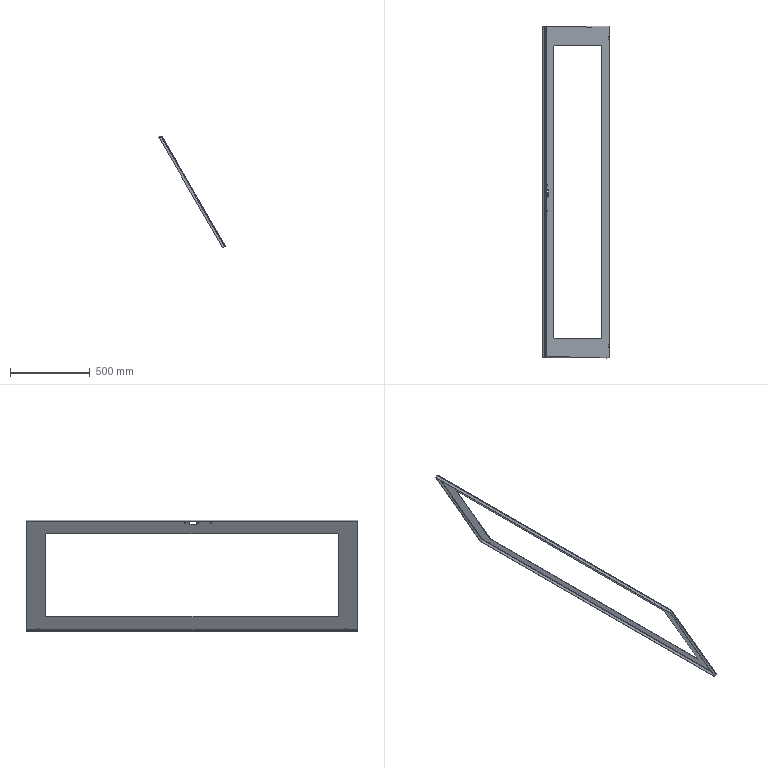Component | SolidWorks | FrontDoorAssembly-1_FrontDoor-1 | 1 solid | 74 faces | volume 1302706 mm3 | plane 40 | cylinder 26 | spline 8 | commonest cylinder face diameters 3.2 x8 5.5 x6 7 x4 11 x4 20 x4 | material Malleable Cast Iron